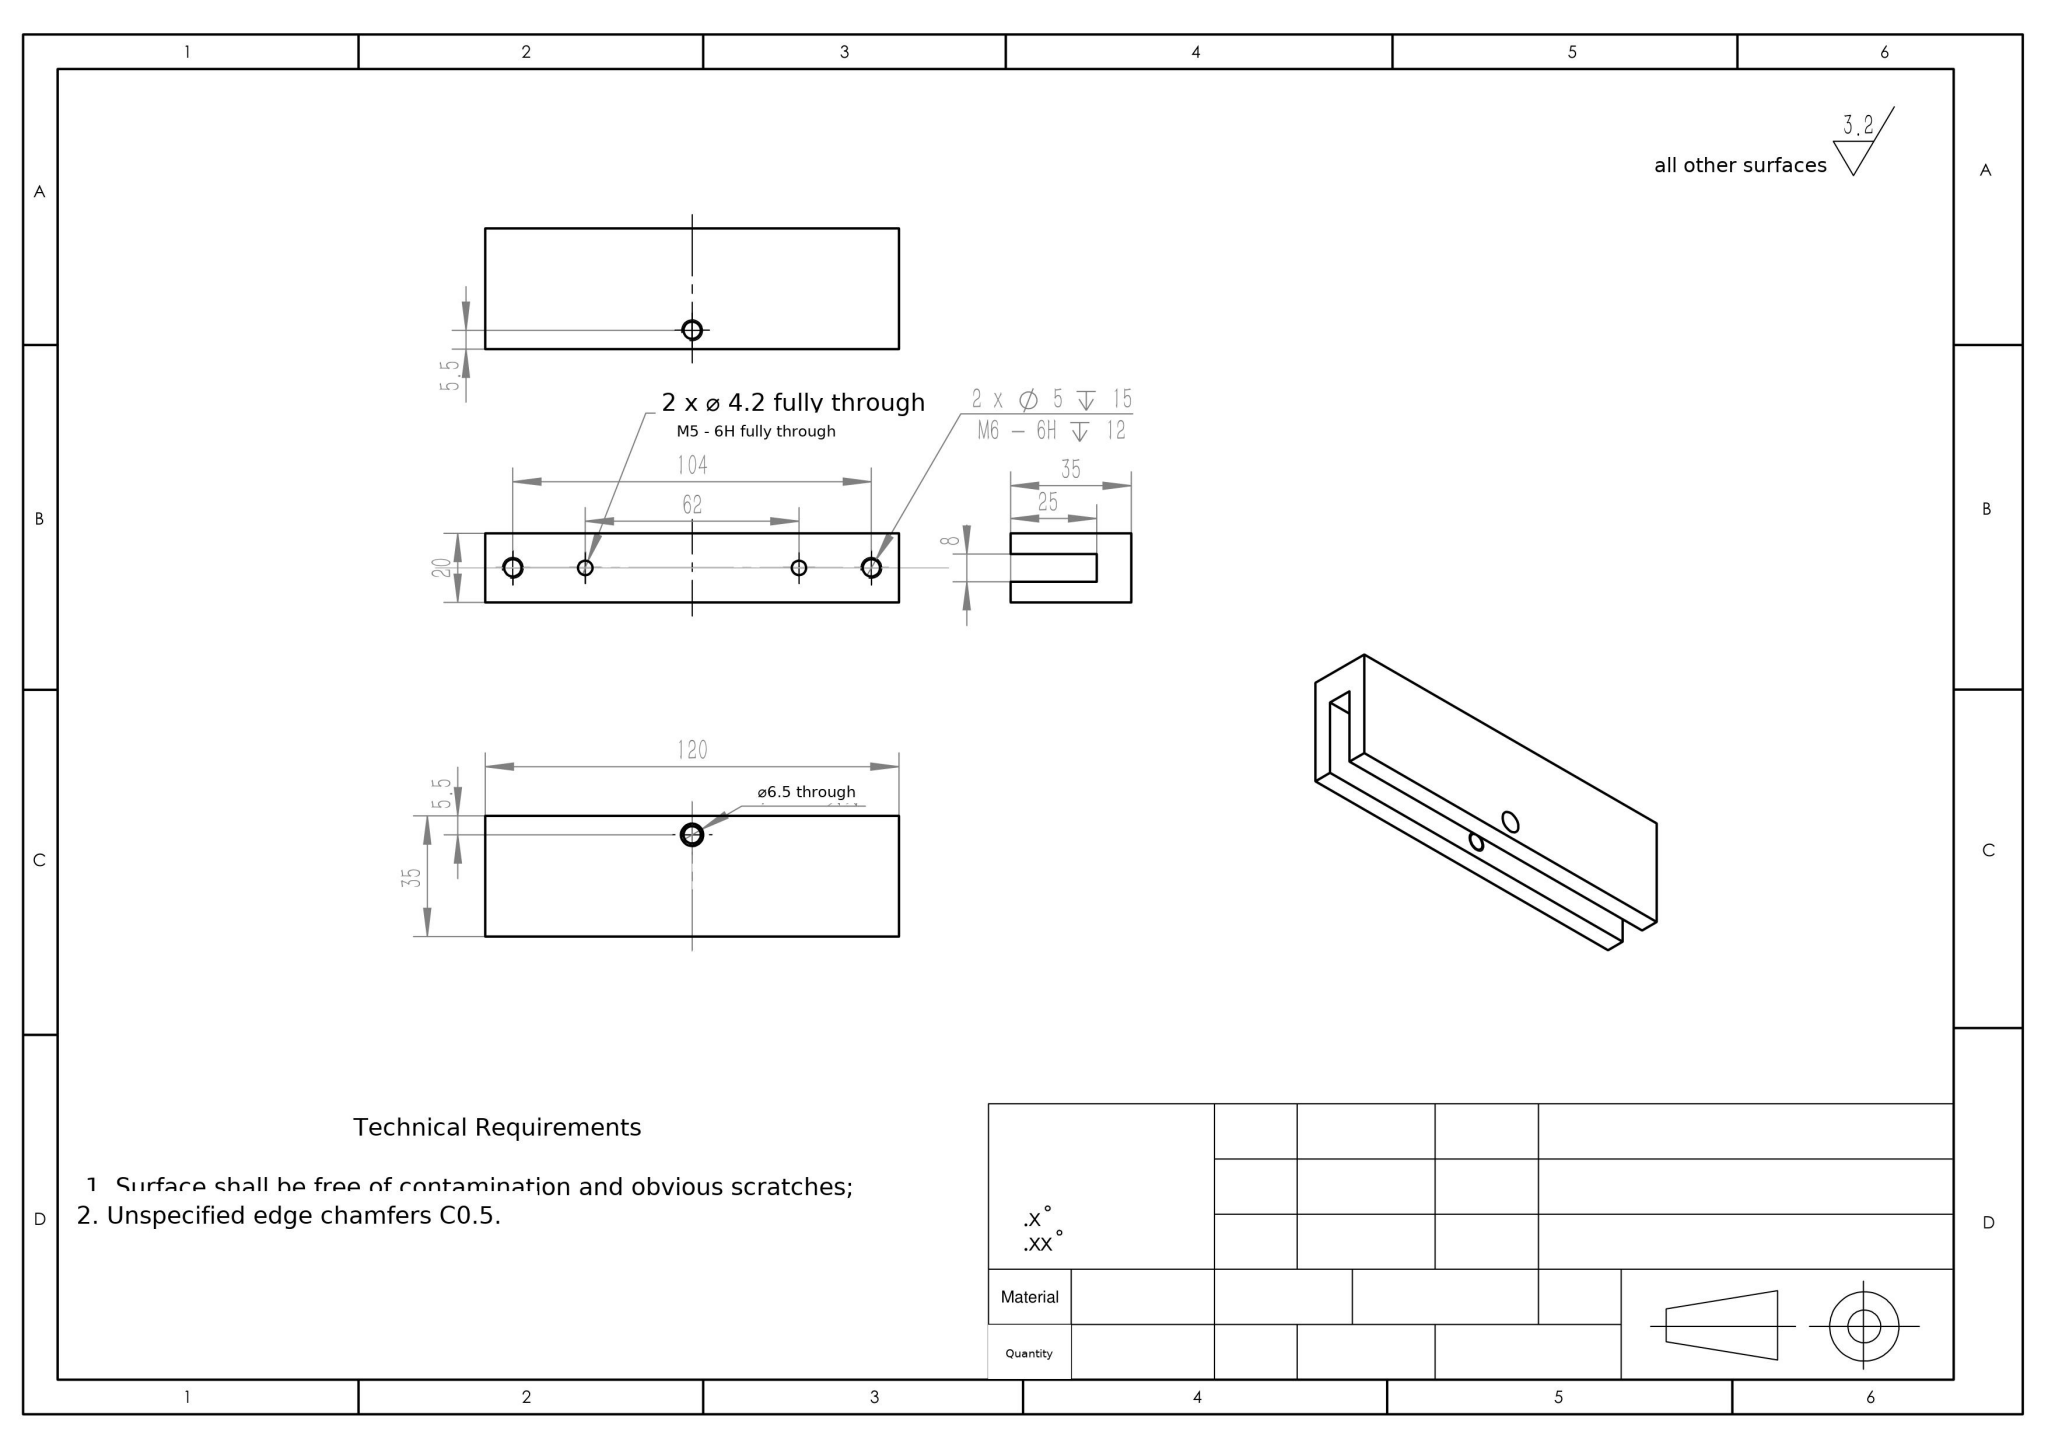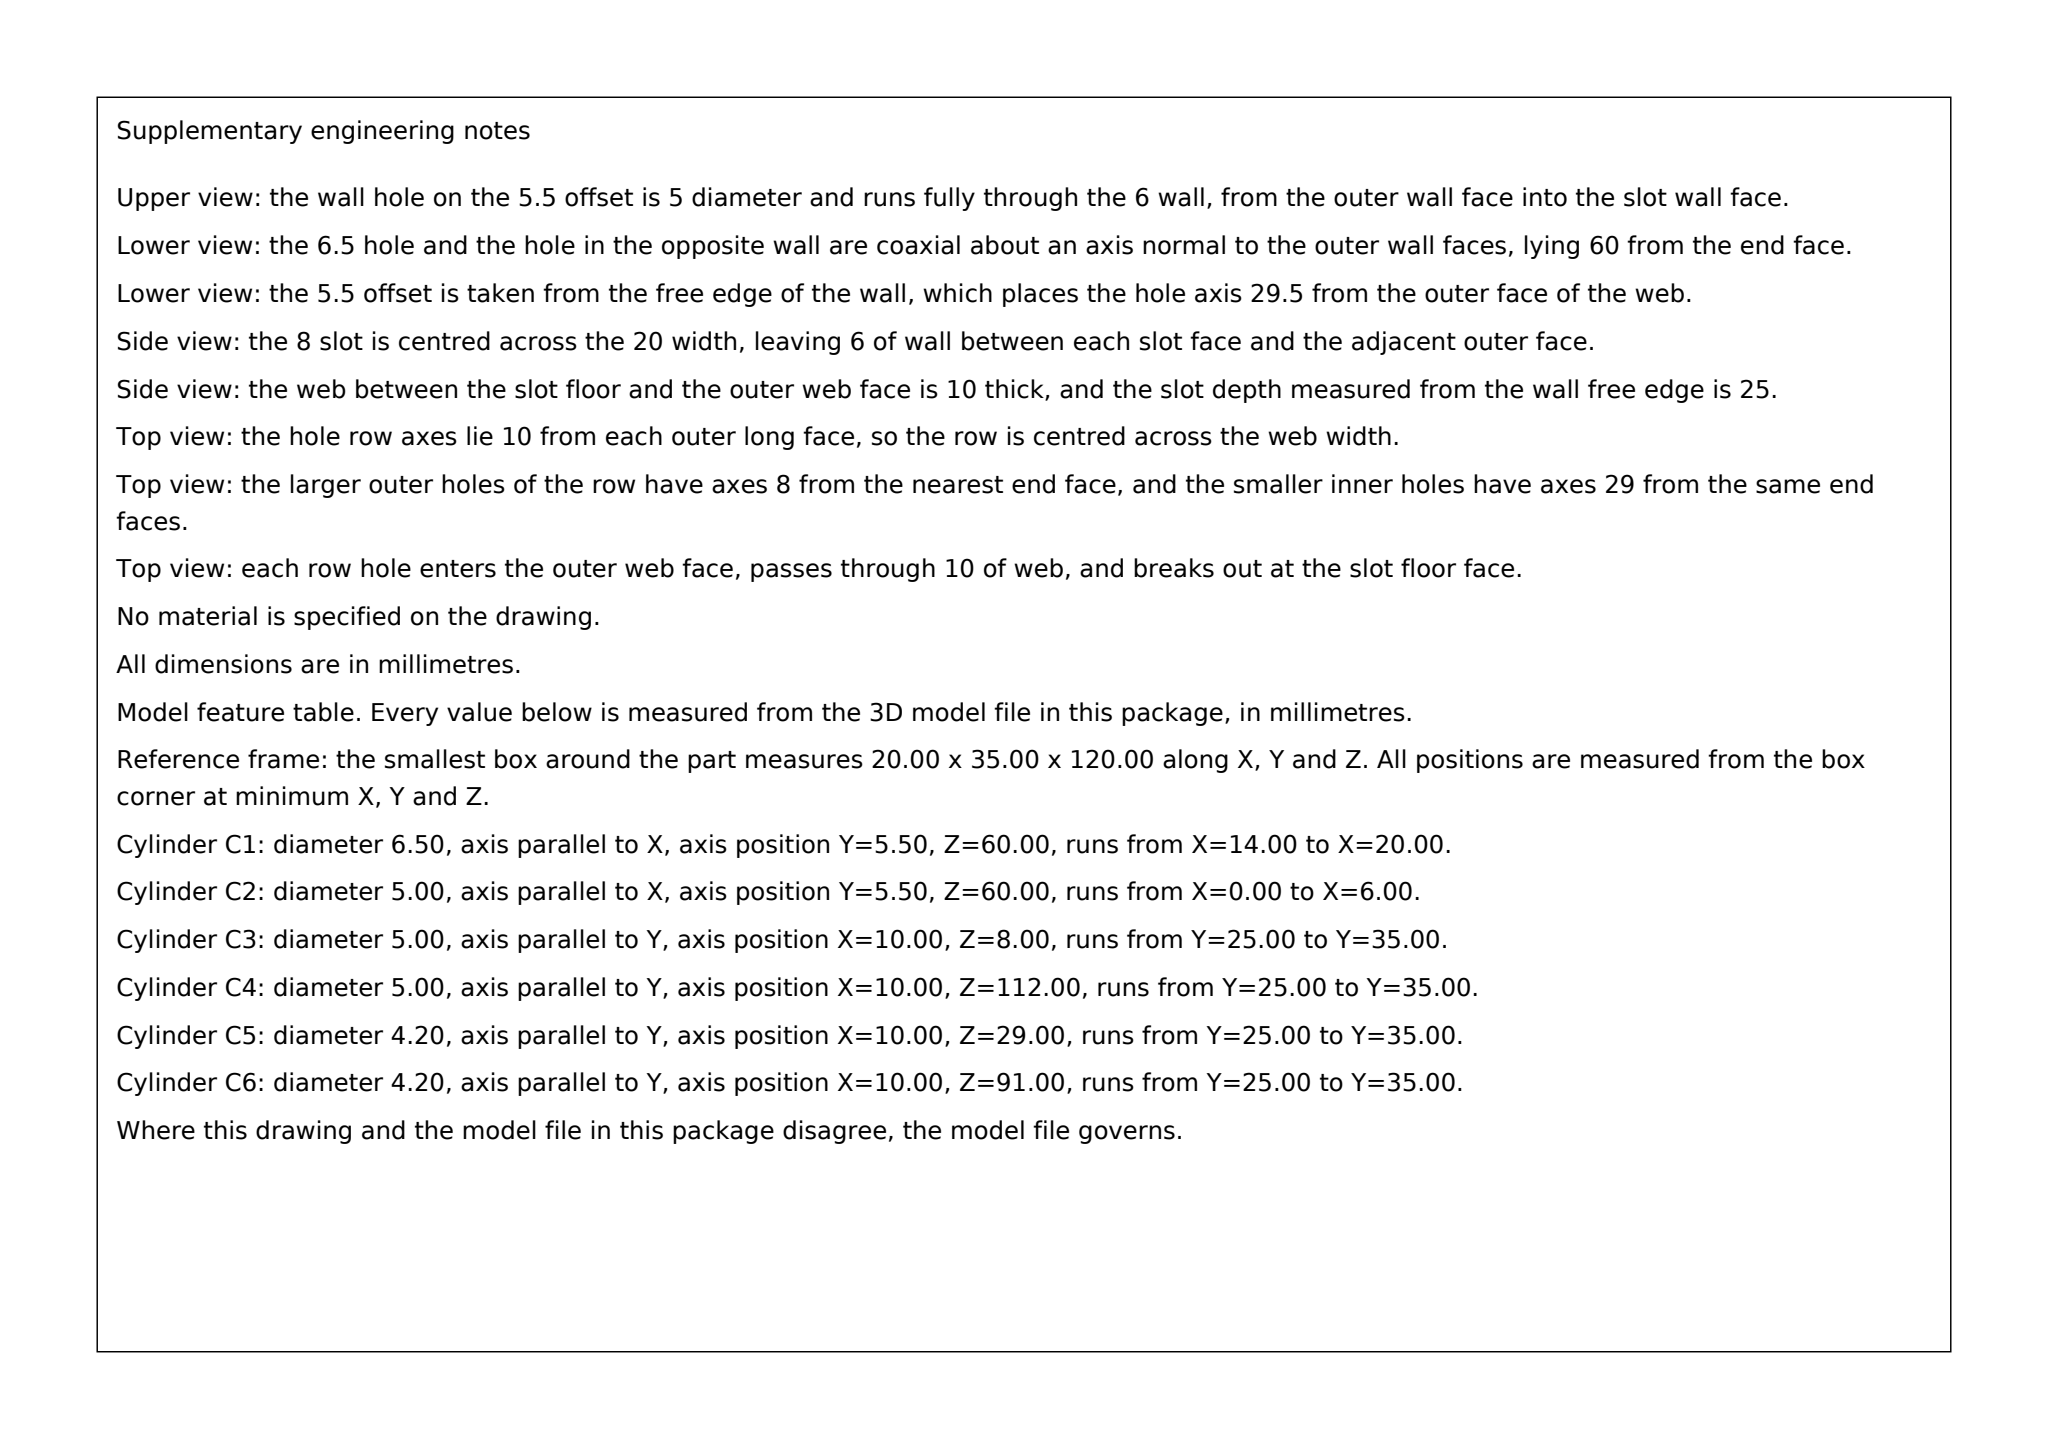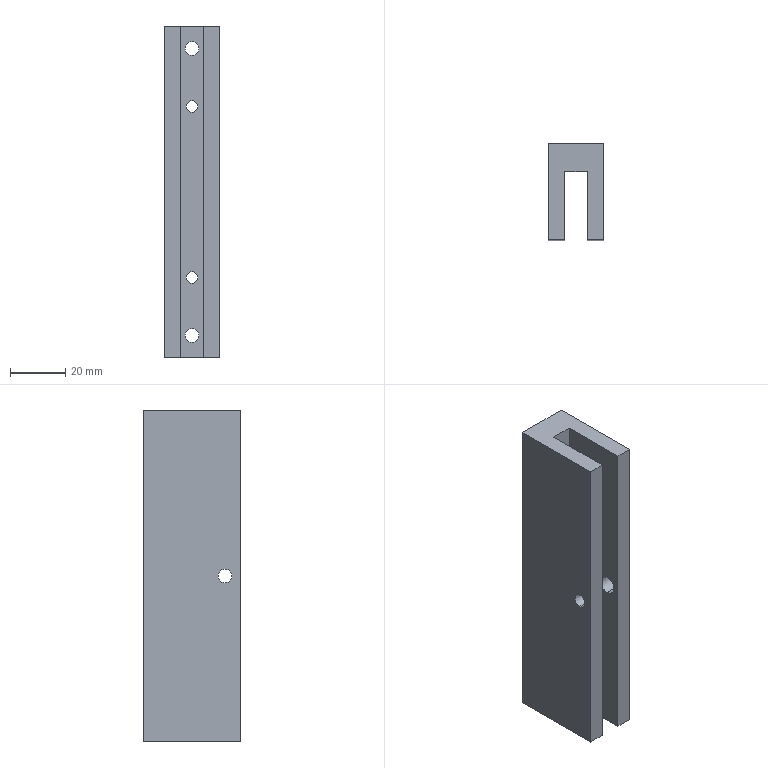Part | SolidWorks | mm | 1 solid | 22 faces | box 20 x 35 x 120 mm | volume 59013 mm3 | cylinder 12 | plane 10 | commonest cylinder face diameters 5 x6 4.2 x4 6.5 x2
build123d program:
from build123d import *

# Parameters (mm, degrees)
BOSS_EXTRUDE1_DEPTH   = 60
M5_TAPPED_HOLE1_D     = 4.2
M6_TAPPED_HOLE1_D     = 5
M6_TAPPED_HOLE1_DEPTH = 15
M6_TAPPED_HOLE1_TIP   = 1.502
CUT_EXTRUDE1_REACH    = 74.284
SKETCH6_R             = 3.25
M6_TAPPED_HOLE2_D     = 5
M6_TAPPED_HOLE2_DEPTH = 15
M6_TAPPED_HOLE2_TIP   = 1.502


with BuildPart() as part:
    # Sketch1 → Boss-Extrude1 (new, symmetric)
    with BuildSketch(Plane.XY):
        Polygon((20, 0), (0, 0), (0, -35), (6, -35), (6, -10), (14, -10), (14, -35), (20, -35), align=None)
    extrude(amount=BOSS_EXTRUDE1_DEPTH, both=True)

    # M5 Tapped Hole1 (through all)
    with Locations(Plane(origin=(0, -10, 0), x_dir=(-1, 0, 0), z_dir=(0, -1, 0))):
        with Locations((-10, -31), (-10, 31)):
            Hole(M5_TAPPED_HOLE1_D / 2)

    # M6 Tapped Hole1
    with Locations(Plane(origin=(0, 0, 0), x_dir=(1, 0, 0), z_dir=(0, 1, 0))):
        with Locations((10, 52), (10, -52)):
            Hole(M6_TAPPED_HOLE1_D / 2, depth=M6_TAPPED_HOLE1_DEPTH)
            with Locations((0, 0, -(M6_TAPPED_HOLE1_DEPTH + M6_TAPPED_HOLE1_TIP / 2))):  # 118° drill point
                Cone(0, M6_TAPPED_HOLE1_D / 2, M6_TAPPED_HOLE1_TIP, mode=Mode.SUBTRACT)

    # Sketch6 → Cut-Extrude1 (cut, up to next)
    with BuildSketch(Plane(origin=(20, 0, 0), x_dir=(0, 0, -1), z_dir=(1, 0, 0)), mode=Mode.PRIVATE) as cut_extrude1_sk1:
        with Locations((0, -29.5)):
            Circle(SKETCH6_R)
    cut_extrude1_tool1 = extrude(cut_extrude1_sk1.sketch, amount=-CUT_EXTRUDE1_REACH, mode=Mode.PRIVATE) & part.part
    add(cut_extrude1_tool1.solids().sort_by_distance((20, -29.5, 0))[0], mode=Mode.SUBTRACT)

    # M6 Tapped Hole2
    with Locations(Plane(origin=(6, 0, 0), x_dir=(0, 0, -1), z_dir=(1, 0, 0))):
        with Locations((0, -29.5)):
            Hole(M6_TAPPED_HOLE2_D / 2, depth=M6_TAPPED_HOLE2_DEPTH)
            with Locations((0, 0, -(M6_TAPPED_HOLE2_DEPTH + M6_TAPPED_HOLE2_TIP / 2))):  # 118° drill point
                Cone(0, M6_TAPPED_HOLE2_D / 2, M6_TAPPED_HOLE2_TIP, mode=Mode.SUBTRACT)


solid = part.part
STEP:
#1=CARTESIAN_POINT('',(0.,-29.5,2.5));
#2=VERTEX_POINT('',#1);
#3=CARTESIAN_POINT('',(0.,-29.5,-2.5));
#4=VERTEX_POINT('',#3);
#5=CARTESIAN_POINT('',(0.,-29.5,-0.));
#6=DIRECTION('',(1.,0.,0.));
#7=DIRECTION('',(0.,0.,-1.));
#8=AXIS2_PLACEMENT_3D('',#5,#6,#7);
#9=CIRCLE('',#8,2.5);
#10=EDGE_CURVE('',#2,#4,#9,.T.);
#11=ORIENTED_EDGE('',*,*,#10,.F.);
#12=CARTESIAN_POINT('',(6.,-29.5,2.5));
#13=VERTEX_POINT('',#12);
#14=CARTESIAN_POINT('',(6.,-29.5,2.5));
#15=DIRECTION('',(1.,0.,0.));
#16=VECTOR('',#15,1000.);
#17=LINE('',#14,#16);
#18=EDGE_CURVE('',#2,#13,#17,.T.);
#19=ORIENTED_EDGE('',*,*,#18,.T.);
#20=CARTESIAN_POINT('',(6.,-29.5,-2.5));
#21=VERTEX_POINT('',#20);
#22=CARTESIAN_POINT('',(6.,-29.5,-0.));
#23=DIRECTION('',(1.,0.,0.));
#24=DIRECTION('',(0.,0.,-1.));
#25=AXIS2_PLACEMENT_3D('',#22,#23,#24);
#26=CIRCLE('',#25,2.5);
#27=EDGE_CURVE('',#13,#21,#26,.T.);
#28=ORIENTED_EDGE('',*,*,#27,.T.);
#29=CARTESIAN_POINT('',(6.,-29.5,-2.5));
#30=DIRECTION('',(1.,0.,0.));
#31=VECTOR('',#30,1000.);
#32=LINE('',#29,#31);
#33=EDGE_CURVE('',#4,#21,#32,.T.);
#34=ORIENTED_EDGE('',*,*,#33,.F.);
#35=EDGE_LOOP('',(#11,#19,#28,#34));
#36=FACE_OUTER_BOUND('',#35,.T.);
#37=CARTESIAN_POINT('',(6.,-29.5,-0.));
#38=DIRECTION('',(1.,0.,0.));
#39=DIRECTION('',(0.,0.,-1.));
#40=AXIS2_PLACEMENT_3D('',#37,#38,#39);
#41=CYLINDRICAL_SURFACE('',#40,2.5);
#42=ADVANCED_FACE('',(#36),#41,.F.);
#43=CARTESIAN_POINT('',(14.,-29.5,-3.25));
#44=VERTEX_POINT('',#43);
#45=CARTESIAN_POINT('',(14.,-29.5,3.25));
#46=VERTEX_POINT('',#45);
#47=CARTESIAN_POINT('',(14.,-29.5,-0.));
#48=DIRECTION('',(-1.,-0.,0.));
#49=DIRECTION('',(0.,1.,0.));
#50=AXIS2_PLACEMENT_3D('',#47,#48,#49);
#51=CIRCLE('',#50,3.25);
#52=EDGE_CURVE('',#44,#46,#51,.T.);
#53=ORIENTED_EDGE('',*,*,#52,.T.);
#54=CARTESIAN_POINT('',(20.,-29.5,3.25));
#55=VERTEX_POINT('',#54);
#56=CARTESIAN_POINT('',(-0.001,-29.5,3.25));
#57=DIRECTION('',(1.,0.,0.));
#58=VECTOR('',#57,1000.);
#59=LINE('',#56,#58);
#60=EDGE_CURVE('',#46,#55,#59,.T.);
#61=ORIENTED_EDGE('',*,*,#60,.T.);
#62=CARTESIAN_POINT('',(20.,-29.5,-3.25));
#63=VERTEX_POINT('',#62);
#64=CARTESIAN_POINT('',(20.,-29.5,-0.));
#65=DIRECTION('',(1.,0.,0.));
#66=DIRECTION('',(0.,0.,-1.));
#67=AXIS2_PLACEMENT_3D('',#64,#65,#66);
#68=CIRCLE('',#67,3.25);
#69=EDGE_CURVE('',#55,#63,#68,.T.);
#70=ORIENTED_EDGE('',*,*,#69,.T.);
#71=CARTESIAN_POINT('',(-0.001,-29.5,-3.25));
#72=DIRECTION('',(1.,0.,0.));
#73=VECTOR('',#72,1000.);
#74=LINE('',#71,#73);
#75=EDGE_CURVE('',#44,#63,#74,.T.);
#76=ORIENTED_EDGE('',*,*,#75,.F.);
#77=EDGE_LOOP('',(#53,#61,#70,#76));
#78=FACE_OUTER_BOUND('',#77,.T.);
#79=CARTESIAN_POINT('',(-0.001,-29.5,-0.));
#80=DIRECTION('',(1.,0.,0.));
#81=DIRECTION('',(0.,0.,-1.));
#82=AXIS2_PLACEMENT_3D('',#79,#80,#81);
#83=CYLINDRICAL_SURFACE('',#82,3.25);
#84=ADVANCED_FACE('',(#78),#83,.F.);
#85=CARTESIAN_POINT('',(10.,-10.,-54.5));
#86=VERTEX_POINT('',#85);
#87=CARTESIAN_POINT('',(10.,-10.,-49.5));
#88=VERTEX_POINT('',#87);
#89=CARTESIAN_POINT('',(10.,-10.,-52.));
#90=DIRECTION('',(0.,1.,0.));
#91=DIRECTION('',(0.,0.,1.));
#92=AXIS2_PLACEMENT_3D('',#89,#90,#91);
#93=CIRCLE('',#92,2.5);
#94=EDGE_CURVE('',#86,#88,#93,.T.);
#95=ORIENTED_EDGE('',*,*,#94,.F.);
#96=CARTESIAN_POINT('',(10.,0.,-54.5));
#97=VERTEX_POINT('',#96);
#98=CARTESIAN_POINT('',(10.,0.,-54.5));
#99=DIRECTION('',(0.,1.,0.));
#100=VECTOR('',#99,1000.);
#101=LINE('',#98,#100);
#102=EDGE_CURVE('',#86,#97,#101,.T.);
#103=ORIENTED_EDGE('',*,*,#102,.T.);
#104=CARTESIAN_POINT('',(10.,0.,-49.5));
#105=VERTEX_POINT('',#104);
#106=CARTESIAN_POINT('',(10.,0.,-52.));
#107=DIRECTION('',(0.,1.,0.));
#108=DIRECTION('',(0.,0.,1.));
#109=AXIS2_PLACEMENT_3D('',#106,#107,#108);
#110=CIRCLE('',#109,2.5);
#111=EDGE_CURVE('',#97,#105,#110,.T.);
#112=ORIENTED_EDGE('',*,*,#111,.T.);
#113=CARTESIAN_POINT('',(10.,0.,-49.5));
#114=DIRECTION('',(0.,1.,0.));
#115=VECTOR('',#114,1000.);
#116=LINE('',#113,#115);
#117=EDGE_CURVE('',#88,#105,#116,.T.);
#118=ORIENTED_EDGE('',*,*,#117,.F.);
#119=EDGE_LOOP('',(#95,#103,#112,#118));
#120=FACE_OUTER_BOUND('',#119,.T.);
#121=CARTESIAN_POINT('',(10.,0.,-52.));
#122=DIRECTION('',(0.,1.,0.));
#123=DIRECTION('',(0.,0.,1.));
#124=AXIS2_PLACEMENT_3D('',#121,#122,#123);
#125=CYLINDRICAL_SURFACE('',#124,2.5);
#126=ADVANCED_FACE('',(#120),#125,.F.);
#127=CARTESIAN_POINT('',(10.,-10.,49.5));
#128=VERTEX_POINT('',#127);
#129=CARTESIAN_POINT('',(10.,-10.,54.5));
#130=VERTEX_POINT('',#129);
#131=CARTESIAN_POINT('',(10.,-10.,52.));
#132=DIRECTION('',(0.,1.,0.));
#133=DIRECTION('',(0.,0.,1.));
#134=AXIS2_PLACEMENT_3D('',#131,#132,#133);
#135=CIRCLE('',#134,2.5);
#136=EDGE_CURVE('',#128,#130,#135,.T.);
#137=ORIENTED_EDGE('',*,*,#136,.F.);
#138=CARTESIAN_POINT('',(10.,0.,49.5));
#139=VERTEX_POINT('',#138);
#140=CARTESIAN_POINT('',(10.,0.,49.5));
#141=DIRECTION('',(0.,1.,0.));
#142=VECTOR('',#141,1000.);
#143=LINE('',#140,#142);
#144=EDGE_CURVE('',#128,#139,#143,.T.);
#145=ORIENTED_EDGE('',*,*,#144,.T.);
#146=CARTESIAN_POINT('',(10.,0.,54.5));
#147=VERTEX_POINT('',#146);
#148=CARTESIAN_POINT('',(10.,0.,52.));
#149=DIRECTION('',(0.,1.,0.));
#150=DIRECTION('',(0.,0.,1.));
#151=AXIS2_PLACEMENT_3D('',#148,#149,#150);
#152=CIRCLE('',#151,2.5);
#153=EDGE_CURVE('',#139,#147,#152,.T.);
#154=ORIENTED_EDGE('',*,*,#153,.T.);
#155=CARTESIAN_POINT('',(10.,0.,54.5));
#156=DIRECTION('',(0.,1.,0.));
#157=VECTOR('',#156,1000.);
#158=LINE('',#155,#157);
#159=EDGE_CURVE('',#130,#147,#158,.T.);
#160=ORIENTED_EDGE('',*,*,#159,.F.);
#161=EDGE_LOOP('',(#137,#145,#154,#160));
#162=FACE_OUTER_BOUND('',#161,.T.);
#163=CARTESIAN_POINT('',(10.,0.,52.));
#164=DIRECTION('',(0.,1.,0.));
#165=DIRECTION('',(0.,0.,1.));
#166=AXIS2_PLACEMENT_3D('',#163,#164,#165);
#167=CYLINDRICAL_SURFACE('',#166,2.5);
#168=ADVANCED_FACE('',(#162),#167,.F.);
#169=CARTESIAN_POINT('',(10.,0.,33.1));
#170=VERTEX_POINT('',#169);
#171=CARTESIAN_POINT('',(10.,0.,28.9));
#172=VERTEX_POINT('',#171);
#173=CARTESIAN_POINT('',(10.,0.,31.));
#174=DIRECTION('',(0.,-1.,0.));
#175=DIRECTION('',(0.,0.,-1.));
#176=AXIS2_PLACEMENT_3D('',#173,#174,#175);
#177=CIRCLE('',#176,2.1);
#178=EDGE_CURVE('',#170,#172,#177,.T.);
#179=ORIENTED_EDGE('',*,*,#178,.F.);
#180=CARTESIAN_POINT('',(10.,-10.,33.1));
#181=VERTEX_POINT('',#180);
#182=CARTESIAN_POINT('',(10.,-10.,33.1));
#183=DIRECTION('',(0.,-1.,0.));
#184=VECTOR('',#183,1000.);
#185=LINE('',#182,#184);
#186=EDGE_CURVE('',#170,#181,#185,.T.);
#187=ORIENTED_EDGE('',*,*,#186,.T.);
#188=CARTESIAN_POINT('',(10.,-10.,28.9));
#189=VERTEX_POINT('',#188);
#190=CARTESIAN_POINT('',(10.,-10.,31.));
#191=DIRECTION('',(0.,-1.,0.));
#192=DIRECTION('',(0.,0.,-1.));
#193=AXIS2_PLACEMENT_3D('',#190,#191,#192);
#194=CIRCLE('',#193,2.1);
#195=EDGE_CURVE('',#181,#189,#194,.T.);
#196=ORIENTED_EDGE('',*,*,#195,.T.);
#197=CARTESIAN_POINT('',(10.,-10.,28.9));
#198=DIRECTION('',(0.,-1.,0.));
#199=VECTOR('',#198,1000.);
#200=LINE('',#197,#199);
#201=EDGE_CURVE('',#172,#189,#200,.T.);
#202=ORIENTED_EDGE('',*,*,#201,.F.);
#203=EDGE_LOOP('',(#179,#187,#196,#202));
#204=FACE_OUTER_BOUND('',#203,.T.);
#205=CARTESIAN_POINT('',(10.,-10.,31.));
#206=DIRECTION('',(0.,-1.,0.));
#207=DIRECTION('',(0.,0.,-1.));
#208=AXIS2_PLACEMENT_3D('',#205,#206,#207);
#209=CYLINDRICAL_SURFACE('',#208,2.1);
#210=ADVANCED_FACE('',(#204),#209,.F.);
#211=CARTESIAN_POINT('',(10.,0.,-28.9));
#212=VERTEX_POINT('',#211);
#213=CARTESIAN_POINT('',(10.,0.,-33.1));
#214=VERTEX_POINT('',#213);
#215=CARTESIAN_POINT('',(10.,0.,-31.));
#216=DIRECTION('',(0.,-1.,0.));
#217=DIRECTION('',(0.,0.,-1.));
#218=AXIS2_PLACEMENT_3D('',#215,#216,#217);
#219=CIRCLE('',#218,2.1);
#220=EDGE_CURVE('',#212,#214,#219,.T.);
#221=ORIENTED_EDGE('',*,*,#220,.F.);
#222=CARTESIAN_POINT('',(10.,-10.,-28.9));
#223=VERTEX_POINT('',#222);
#224=CARTESIAN_POINT('',(10.,-10.,-28.9));
#225=DIRECTION('',(0.,-1.,0.));
#226=VECTOR('',#225,1000.);
#227=LINE('',#224,#226);
#228=EDGE_CURVE('',#212,#223,#227,.T.);
#229=ORIENTED_EDGE('',*,*,#228,.T.);
#230=CARTESIAN_POINT('',(10.,-10.,-33.1));
#231=VERTEX_POINT('',#230);
#232=CARTESIAN_POINT('',(10.,-10.,-31.));
#233=DIRECTION('',(0.,-1.,0.));
#234=DIRECTION('',(0.,0.,-1.));
#235=AXIS2_PLACEMENT_3D('',#232,#233,#234);
#236=CIRCLE('',#235,2.1);
#237=EDGE_CURVE('',#223,#231,#236,.T.);
#238=ORIENTED_EDGE('',*,*,#237,.T.);
#239=CARTESIAN_POINT('',(10.,-10.,-33.1));
#240=DIRECTION('',(0.,-1.,0.));
#241=VECTOR('',#240,1000.);
#242=LINE('',#239,#241);
#243=EDGE_CURVE('',#214,#231,#242,.T.);
#244=ORIENTED_EDGE('',*,*,#243,.F.);
#245=EDGE_LOOP('',(#221,#229,#238,#244));
#246=FACE_OUTER_BOUND('',#245,.T.);
#247=CARTESIAN_POINT('',(10.,-10.,-31.));
#248=DIRECTION('',(0.,-1.,0.));
#249=DIRECTION('',(0.,0.,-1.));
#250=AXIS2_PLACEMENT_3D('',#247,#248,#249);
#251=CYLINDRICAL_SURFACE('',#250,2.1);
#252=ADVANCED_FACE('',(#246),#251,.F.);
#253=CARTESIAN_POINT('',(20.,-29.5,-0.));
#254=DIRECTION('',(1.,0.,0.));
#255=DIRECTION('',(0.,0.,-1.));
#256=AXIS2_PLACEMENT_3D('',#253,#254,#255);
#257=CIRCLE('',#256,3.25);
#258=EDGE_CURVE('',#63,#55,#257,.T.);
#259=ORIENTED_EDGE('',*,*,#258,.F.);
#260=ORIENTED_EDGE('',*,*,#69,.F.);
#261=EDGE_LOOP('',(#259,#260));
#262=FACE_BOUND('',#261,.T.);
#263=CARTESIAN_POINT('',(20.,-35.,-60.));
#264=VERTEX_POINT('',#263);
#265=CARTESIAN_POINT('',(20.,-0.,-60.));
#266=VERTEX_POINT('',#265);
#267=CARTESIAN_POINT('',(20.,-35.,-60.));
#268=DIRECTION('',(0.,1.,0.));
#269=VECTOR('',#268,1000.);
#270=LINE('',#267,#269);
#271=EDGE_CURVE('',#264,#266,#270,.T.);
#272=ORIENTED_EDGE('',*,*,#271,.T.);
#273=CARTESIAN_POINT('',(20.,-0.,60.));
#274=VERTEX_POINT('',#273);
#275=CARTESIAN_POINT('',(20.,-0.,60.));
#276=DIRECTION('',(0.,0.,-1.));
#277=VECTOR('',#276,1000.);
#278=LINE('',#275,#277);
#279=EDGE_CURVE('',#274,#266,#278,.T.);
#280=ORIENTED_EDGE('',*,*,#279,.F.);
#281=CARTESIAN_POINT('',(20.,-35.,60.));
#282=VERTEX_POINT('',#281);
#283=CARTESIAN_POINT('',(20.,-35.,60.));
#284=DIRECTION('',(0.,1.,0.));
#285=VECTOR('',#284,1000.);
#286=LINE('',#283,#285);
#287=EDGE_CURVE('',#282,#274,#286,.T.);
#288=ORIENTED_EDGE('',*,*,#287,.F.);
#289=CARTESIAN_POINT('',(20.,-35.,60.));
#290=DIRECTION('',(0.,0.,-1.));
#291=VECTOR('',#290,1000.);
#292=LINE('',#289,#291);
#293=EDGE_CURVE('',#282,#264,#292,.T.);
#294=ORIENTED_EDGE('',*,*,#293,.T.);
#295=EDGE_LOOP('',(#272,#280,#288,#294));
#296=FACE_OUTER_BOUND('',#295,.T.);
#297=CARTESIAN_POINT('',(20.,-35.,60.));
#298=DIRECTION('',(-1.,0.,0.));
#299=DIRECTION('',(0.,0.,1.));
#300=AXIS2_PLACEMENT_3D('',#297,#298,#299);
#301=PLANE('',#300);
#302=ADVANCED_FACE('',(#262,#296),#301,.F.);
#303=CARTESIAN_POINT('',(10.,0.,-52.));
#304=DIRECTION('',(0.,1.,0.));
#305=DIRECTION('',(0.,0.,1.));
#306=AXIS2_PLACEMENT_3D('',#303,#304,#305);
#307=CIRCLE('',#306,2.5);
#308=EDGE_CURVE('',#105,#97,#307,.T.);
#309=ORIENTED_EDGE('',*,*,#308,.F.);
#310=ORIENTED_EDGE('',*,*,#111,.F.);
#311=EDGE_LOOP('',(#309,#310));
#312=FACE_BOUND('',#311,.T.);
#313=CARTESIAN_POINT('',(10.,0.,52.));
#314=DIRECTION('',(0.,1.,0.));
#315=DIRECTION('',(0.,0.,1.));
#316=AXIS2_PLACEMENT_3D('',#313,#314,#315);
#317=CIRCLE('',#316,2.5);
#318=EDGE_CURVE('',#147,#139,#317,.T.);
#319=ORIENTED_EDGE('',*,*,#318,.F.);
#320=ORIENTED_EDGE('',*,*,#153,.F.);
#321=EDGE_LOOP('',(#319,#320));
#322=FACE_BOUND('',#321,.T.);
#323=CARTESIAN_POINT('',(10.,0.,31.));
#324=DIRECTION('',(0.,-1.,0.));
#325=DIRECTION('',(0.,0.,-1.));
#326=AXIS2_PLACEMENT_3D('',#323,#324,#325);
#327=CIRCLE('',#326,2.1);
#328=EDGE_CURVE('',#172,#170,#327,.T.);
#329=ORIENTED_EDGE('',*,*,#328,.T.);
#330=ORIENTED_EDGE('',*,*,#178,.T.);
#331=EDGE_LOOP('',(#329,#330));
#332=FACE_BOUND('',#331,.T.);
#333=CARTESIAN_POINT('',(10.,0.,-31.));
#334=DIRECTION('',(0.,-1.,0.));
#335=DIRECTION('',(0.,0.,-1.));
#336=AXIS2_PLACEMENT_3D('',#333,#334,#335);
#337=CIRCLE('',#336,2.1);
#338=EDGE_CURVE('',#214,#212,#337,.T.);
#339=ORIENTED_EDGE('',*,*,#338,.T.);
#340=ORIENTED_EDGE('',*,*,#220,.T.);
#341=EDGE_LOOP('',(#339,#340));
#342=FACE_BOUND('',#341,.T.);
#343=CARTESIAN_POINT('',(0.,0.,-60.));
#344=VERTEX_POINT('',#343);
#345=CARTESIAN_POINT('',(20.,-0.,-60.));
#346=DIRECTION('',(-1.,0.,0.));
#347=VECTOR('',#346,1000.);
#348=LINE('',#345,#347);
#349=EDGE_CURVE('',#266,#344,#348,.T.);
#350=ORIENTED_EDGE('',*,*,#349,.T.);
#351=CARTESIAN_POINT('',(0.,0.,60.));
#352=VERTEX_POINT('',#351);
#353=CARTESIAN_POINT('',(0.,0.,60.));
#354=DIRECTION('',(0.,0.,-1.));
#355=VECTOR('',#354,1000.);
#356=LINE('',#353,#355);
#357=EDGE_CURVE('',#352,#344,#356,.T.);
#358=ORIENTED_EDGE('',*,*,#357,.F.);
#359=CARTESIAN_POINT('',(20.,-0.,60.));
#360=DIRECTION('',(-1.,0.,0.));
#361=VECTOR('',#360,1000.);
#362=LINE('',#359,#361);
#363=EDGE_CURVE('',#274,#352,#362,.T.);
#364=ORIENTED_EDGE('',*,*,#363,.F.);
#365=ORIENTED_EDGE('',*,*,#279,.T.);
#366=EDGE_LOOP('',(#350,#358,#364,#365));
#367=FACE_OUTER_BOUND('',#366,.T.);
#368=CARTESIAN_POINT('',(20.,-0.,60.));
#369=DIRECTION('',(-0.,-1.,0.));
#370=DIRECTION('',(1.,-0.,0.));
#371=AXIS2_PLACEMENT_3D('',#368,#369,#370);
#372=PLANE('',#371);
#373=ADVANCED_FACE('',(#312,#322,#332,#342,#367),#372,.F.);
#374=CARTESIAN_POINT('',(0.,-29.5,-0.));
#375=DIRECTION('',(1.,0.,0.));
#376=DIRECTION('',(0.,0.,-1.));
#377=AXIS2_PLACEMENT_3D('',#374,#375,#376);
#378=CIRCLE('',#377,2.5);
#379=EDGE_CURVE('',#4,#2,#378,.T.);
#380=ORIENTED_EDGE('',*,*,#379,.T.);
#381=ORIENTED_EDGE('',*,*,#10,.T.);
#382=EDGE_LOOP('',(#380,#381));
#383=FACE_BOUND('',#382,.T.);
#384=CARTESIAN_POINT('',(0.,-35.,-60.));
#385=VERTEX_POINT('',#384);
#386=CARTESIAN_POINT('',(0.,0.,-60.));
#387=DIRECTION('',(0.,-1.,0.));
#388=VECTOR('',#387,1000.);
#389=LINE('',#386,#388);
#390=EDGE_CURVE('',#344,#385,#389,.T.);
#391=ORIENTED_EDGE('',*,*,#390,.T.);
#392=CARTESIAN_POINT('',(0.,-35.,60.));
#393=VERTEX_POINT('',#392);
#394=CARTESIAN_POINT('',(0.,-35.,60.));
#395=DIRECTION('',(0.,0.,-1.));
#396=VECTOR('',#395,1000.);
#397=LINE('',#394,#396);
#398=EDGE_CURVE('',#393,#385,#397,.T.);
#399=ORIENTED_EDGE('',*,*,#398,.F.);
#400=CARTESIAN_POINT('',(0.,0.,60.));
#401=DIRECTION('',(0.,-1.,0.));
#402=VECTOR('',#401,1000.);
#403=LINE('',#400,#402);
#404=EDGE_CURVE('',#352,#393,#403,.T.);
#405=ORIENTED_EDGE('',*,*,#404,.F.);
#406=ORIENTED_EDGE('',*,*,#357,.T.);
#407=EDGE_LOOP('',(#391,#399,#405,#406));
#408=FACE_OUTER_BOUND('',#407,.T.);
#409=CARTESIAN_POINT('',(0.,0.,60.));
#410=DIRECTION('',(1.,0.,0.));
#411=DIRECTION('',(0.,0.,-1.));
#412=AXIS2_PLACEMENT_3D('',#409,#410,#411);
#413=PLANE('',#412);
#414=ADVANCED_FACE('',(#383,#408),#413,.F.);
#415=CARTESIAN_POINT('',(6.,-35.,-60.));
#416=VERTEX_POINT('',#415);
#417=CARTESIAN_POINT('',(0.,-35.,-60.));
#418=DIRECTION('',(1.,0.,0.));
#419=VECTOR('',#418,1000.);
#420=LINE('',#417,#419);
#421=EDGE_CURVE('',#385,#416,#420,.T.);
#422=ORIENTED_EDGE('',*,*,#421,.T.);
#423=CARTESIAN_POINT('',(6.,-35.,60.));
#424=VERTEX_POINT('',#423);
#425=CARTESIAN_POINT('',(6.,-35.,60.));
#426=DIRECTION('',(0.,0.,-1.));
#427=VECTOR('',#426,1000.);
#428=LINE('',#425,#427);
#429=EDGE_CURVE('',#424,#416,#428,.T.);
#430=ORIENTED_EDGE('',*,*,#429,.F.);
#431=CARTESIAN_POINT('',(0.,-35.,60.));
#432=DIRECTION('',(1.,0.,0.));
#433=VECTOR('',#432,1000.);
#434=LINE('',#431,#433);
#435=EDGE_CURVE('',#393,#424,#434,.T.);
#436=ORIENTED_EDGE('',*,*,#435,.F.);
#437=ORIENTED_EDGE('',*,*,#398,.T.);
#438=EDGE_LOOP('',(#422,#430,#436,#437));
#439=FACE_OUTER_BOUND('',#438,.T.);
#440=CARTESIAN_POINT('',(0.,-35.,60.));
#441=DIRECTION('',(0.,1.,0.));
#442=DIRECTION('',(0.,0.,1.));
#443=AXIS2_PLACEMENT_3D('',#440,#441,#442);
#444=PLANE('',#443);
#445=ADVANCED_FACE('',(#439),#444,.F.);
#446=CARTESIAN_POINT('',(6.,-29.5,-0.));
#447=DIRECTION('',(1.,0.,0.));
#448=DIRECTION('',(0.,0.,-1.));
#449=AXIS2_PLACEMENT_3D('',#446,#447,#448);
#450=CIRCLE('',#449,2.5);
#451=EDGE_CURVE('',#21,#13,#450,.T.);
#452=ORIENTED_EDGE('',*,*,#451,.F.);
#453=ORIENTED_EDGE('',*,*,#27,.F.);
#454=EDGE_LOOP('',(#452,#453));
#455=FACE_BOUND('',#454,.T.);
#456=CARTESIAN_POINT('',(6.,-10.,-60.));
#457=VERTEX_POINT('',#456);
#458=CARTESIAN_POINT('',(6.,-35.,-60.));
#459=DIRECTION('',(-0.,1.,0.));
#460=VECTOR('',#459,1000.);
#461=LINE('',#458,#460);
#462=EDGE_CURVE('',#416,#457,#461,.T.);
#463=ORIENTED_EDGE('',*,*,#462,.T.);
#464=CARTESIAN_POINT('',(6.,-10.,60.));
#465=VERTEX_POINT('',#464);
#466=CARTESIAN_POINT('',(6.,-10.,60.));
#467=DIRECTION('',(0.,0.,-1.));
#468=VECTOR('',#467,1000.);
#469=LINE('',#466,#468);
#470=EDGE_CURVE('',#465,#457,#469,.T.);
#471=ORIENTED_EDGE('',*,*,#470,.F.);
#472=CARTESIAN_POINT('',(6.,-35.,60.));
#473=DIRECTION('',(-0.,1.,0.));
#474=VECTOR('',#473,1000.);
#475=LINE('',#472,#474);
#476=EDGE_CURVE('',#424,#465,#475,.T.);
#477=ORIENTED_EDGE('',*,*,#476,.F.);
#478=ORIENTED_EDGE('',*,*,#429,.T.);
#479=EDGE_LOOP('',(#463,#471,#477,#478));
#480=FACE_OUTER_BOUND('',#479,.T.);
#481=CARTESIAN_POINT('',(6.,-35.,60.));
#482=DIRECTION('',(-1.,-0.,0.));
#483=DIRECTION('',(0.,-1.,0.));
#484=AXIS2_PLACEMENT_3D('',#481,#482,#483);
#485=PLANE('',#484);
#486=ADVANCED_FACE('',(#455,#480),#485,.F.);
#487=CARTESIAN_POINT('',(10.,-10.,-52.));
#488=DIRECTION('',(0.,1.,0.));
#489=DIRECTION('',(0.,0.,1.));
#490=AXIS2_PLACEMENT_3D('',#487,#488,#489);
#491=CIRCLE('',#490,2.5);
#492=EDGE_CURVE('',#88,#86,#491,.T.);
#493=ORIENTED_EDGE('',*,*,#492,.T.);
#494=ORIENTED_EDGE('',*,*,#94,.T.);
#495=EDGE_LOOP('',(#493,#494));
#496=FACE_BOUND('',#495,.T.);
#497=CARTESIAN_POINT('',(10.,-10.,52.));
#498=DIRECTION('',(0.,1.,0.));
#499=DIRECTION('',(0.,0.,1.));
#500=AXIS2_PLACEMENT_3D('',#497,#498,#499);
#501=CIRCLE('',#500,2.5);
#502=EDGE_CURVE('',#130,#128,#501,.T.);
#503=ORIENTED_EDGE('',*,*,#502,.T.);
#504=ORIENTED_EDGE('',*,*,#136,.T.);
#505=EDGE_LOOP('',(#503,#504));
#506=FACE_BOUND('',#505,.T.);
#507=CARTESIAN_POINT('',(10.,-10.,31.));
#508=DIRECTION('',(0.,-1.,0.));
#509=DIRECTION('',(0.,0.,-1.));
#510=AXIS2_PLACEMENT_3D('',#507,#508,#509);
#511=CIRCLE('',#510,2.1);
#512=EDGE_CURVE('',#189,#181,#511,.T.);
#513=ORIENTED_EDGE('',*,*,#512,.F.);
#514=ORIENTED_EDGE('',*,*,#195,.F.);
#515=EDGE_LOOP('',(#513,#514));
#516=FACE_BOUND('',#515,.T.);
#517=CARTESIAN_POINT('',(10.,-10.,-31.));
#518=DIRECTION('',(0.,-1.,0.));
#519=DIRECTION('',(0.,0.,-1.));
#520=AXIS2_PLACEMENT_3D('',#517,#518,#519);
#521=CIRCLE('',#520,2.1);
#522=EDGE_CURVE('',#231,#223,#521,.T.);
#523=ORIENTED_EDGE('',*,*,#522,.F.);
#524=ORIENTED_EDGE('',*,*,#237,.F.);
#525=EDGE_LOOP('',(#523,#524));
#526=FACE_BOUND('',#525,.T.);
#527=CARTESIAN_POINT('',(14.,-10.,-60.));
#528=VERTEX_POINT('',#527);
#529=CARTESIAN_POINT('',(6.,-10.,-60.));
#530=DIRECTION('',(1.,0.,0.));
#531=VECTOR('',#530,1000.);
#532=LINE('',#529,#531);
#533=EDGE_CURVE('',#457,#528,#532,.T.);
#534=ORIENTED_EDGE('',*,*,#533,.T.);
#535=CARTESIAN_POINT('',(14.,-10.,60.));
#536=VERTEX_POINT('',#535);
#537=CARTESIAN_POINT('',(14.,-10.,60.));
#538=DIRECTION('',(0.,0.,-1.));
#539=VECTOR('',#538,1000.);
#540=LINE('',#537,#539);
#541=EDGE_CURVE('',#536,#528,#540,.T.);
#542=ORIENTED_EDGE('',*,*,#541,.F.);
#543=CARTESIAN_POINT('',(6.,-10.,60.));
#544=DIRECTION('',(1.,0.,0.));
#545=VECTOR('',#544,1000.);
#546=LINE('',#543,#545);
#547=EDGE_CURVE('',#465,#536,#546,.T.);
#548=ORIENTED_EDGE('',*,*,#547,.F.);
#549=ORIENTED_EDGE('',*,*,#470,.T.);
#550=EDGE_LOOP('',(#534,#542,#548,#549));
#551=FACE_OUTER_BOUND('',#550,.T.);
#552=CARTESIAN_POINT('',(6.,-10.,60.));
#553=DIRECTION('',(0.,1.,0.));
#554=DIRECTION('',(0.,0.,1.));
#555=AXIS2_PLACEMENT_3D('',#552,#553,#554);
#556=PLANE('',#555);
#557=ADVANCED_FACE('',(#496,#506,#516,#526,#551),#556,.F.);
#558=ORIENTED_EDGE('',*,*,#52,.F.);
#559=CARTESIAN_POINT('',(14.,-29.5,-0.));
#560=DIRECTION('',(-1.,-0.,0.));
#561=DIRECTION('',(0.,1.,0.));
#562=AXIS2_PLACEMENT_3D('',#559,#560,#561);
#563=CIRCLE('',#562,3.25);
#564=EDGE_CURVE('',#46,#44,#563,.T.);
#565=ORIENTED_EDGE('',*,*,#564,.F.);
#566=EDGE_LOOP('',(#558,#565));
#567=FACE_BOUND('',#566,.T.);
#568=CARTESIAN_POINT('',(14.,-35.,-60.));
#569=VERTEX_POINT('',#568);
#570=CARTESIAN_POINT('',(14.,-10.,-60.));
#571=DIRECTION('',(0.,-1.,0.));
#572=VECTOR('',#571,1000.);
#573=LINE('',#570,#572);
#574=EDGE_CURVE('',#528,#569,#573,.T.);
#575=ORIENTED_EDGE('',*,*,#574,.T.);
#576=CARTESIAN_POINT('',(14.,-35.,60.));
#577=VERTEX_POINT('',#576);
#578=CARTESIAN_POINT('',(14.,-35.,60.));
#579=DIRECTION('',(0.,0.,-1.));
#580=VECTOR('',#579,1000.);
#581=LINE('',#578,#580);
#582=EDGE_CURVE('',#577,#569,#581,.T.);
#583=ORIENTED_EDGE('',*,*,#582,.F.);
#584=CARTESIAN_POINT('',(14.,-10.,60.));
#585=DIRECTION('',(0.,-1.,0.));
#586=VECTOR('',#585,1000.);
#587=LINE('',#584,#586);
#588=EDGE_CURVE('',#536,#577,#587,.T.);
#589=ORIENTED_EDGE('',*,*,#588,.F.);
#590=ORIENTED_EDGE('',*,*,#541,.T.);
#591=EDGE_LOOP('',(#575,#583,#589,#590));
#592=FACE_OUTER_BOUND('',#591,.T.);
#593=CARTESIAN_POINT('',(14.,-10.,60.));
#594=DIRECTION('',(1.,0.,0.));
#595=DIRECTION('',(-0.,1.,0.));
#596=AXIS2_PLACEMENT_3D('',#593,#594,#595);
#597=PLANE('',#596);
#598=ADVANCED_FACE('',(#567,#592),#597,.F.);
#599=CARTESIAN_POINT('',(14.,-35.,-60.));
#600=DIRECTION('',(1.,0.,0.));
#601=VECTOR('',#600,1000.);
#602=LINE('',#599,#601);
#603=EDGE_CURVE('',#569,#264,#602,.T.);
#604=ORIENTED_EDGE('',*,*,#603,.T.);
#605=ORIENTED_EDGE('',*,*,#293,.F.);
#606=CARTESIAN_POINT('',(14.,-35.,60.));
#607=DIRECTION('',(1.,0.,0.));
#608=VECTOR('',#607,1000.);
#609=LINE('',#606,#608);
#610=EDGE_CURVE('',#577,#282,#609,.T.);
#611=ORIENTED_EDGE('',*,*,#610,.F.);
#612=ORIENTED_EDGE('',*,*,#582,.T.);
#613=EDGE_LOOP('',(#604,#605,#611,#612));
#614=FACE_OUTER_BOUND('',#613,.T.);
#615=CARTESIAN_POINT('',(14.,-35.,60.));
#616=DIRECTION('',(0.,1.,0.));
#617=DIRECTION('',(0.,0.,1.));
#618=AXIS2_PLACEMENT_3D('',#615,#616,#617);
#619=PLANE('',#618);
#620=ADVANCED_FACE('',(#614),#619,.F.);
#621=ORIENTED_EDGE('',*,*,#287,.T.);
#622=ORIENTED_EDGE('',*,*,#363,.T.);
#623=ORIENTED_EDGE('',*,*,#404,.T.);
#624=ORIENTED_EDGE('',*,*,#435,.T.);
#625=ORIENTED_EDGE('',*,*,#476,.T.);
#626=ORIENTED_EDGE('',*,*,#547,.T.);
#627=ORIENTED_EDGE('',*,*,#588,.T.);
#628=ORIENTED_EDGE('',*,*,#610,.T.);
#629=EDGE_LOOP('',(#621,#622,#623,#624,#625,#626,#627,#628));
#630=FACE_OUTER_BOUND('',#629,.T.);
#631=CARTESIAN_POINT('',(0.,0.,60.));
#632=DIRECTION('',(0.,0.,1.));
#633=DIRECTION('',(1.,0.,0.));
#634=AXIS2_PLACEMENT_3D('',#631,#632,#633);
#635=PLANE('',#634);
#636=ADVANCED_FACE('',(#630),#635,.T.);
#637=ORIENTED_EDGE('',*,*,#271,.F.);
#638=ORIENTED_EDGE('',*,*,#603,.F.);
#639=ORIENTED_EDGE('',*,*,#574,.F.);
#640=ORIENTED_EDGE('',*,*,#533,.F.);
#641=ORIENTED_EDGE('',*,*,#462,.F.);
#642=ORIENTED_EDGE('',*,*,#421,.F.);
#643=ORIENTED_EDGE('',*,*,#390,.F.);
#644=ORIENTED_EDGE('',*,*,#349,.F.);
#645=EDGE_LOOP('',(#637,#638,#639,#640,#641,#642,#643,#644));
#646=FACE_OUTER_BOUND('',#645,.T.);
#647=CARTESIAN_POINT('',(0.,0.,-60.));
#648=DIRECTION('',(0.,0.,1.));
#649=DIRECTION('',(1.,0.,0.));
#650=AXIS2_PLACEMENT_3D('',#647,#648,#649);
#651=PLANE('',#650);
#652=ADVANCED_FACE('',(#646),#651,.F.);
#653=ORIENTED_EDGE('',*,*,#228,.F.);
#654=ORIENTED_EDGE('',*,*,#338,.F.);
#655=ORIENTED_EDGE('',*,*,#243,.T.);
#656=ORIENTED_EDGE('',*,*,#522,.T.);
#657=EDGE_LOOP('',(#653,#654,#655,#656));
#658=FACE_OUTER_BOUND('',#657,.T.);
#659=CARTESIAN_POINT('',(10.,-10.,-31.));
#660=DIRECTION('',(0.,-1.,0.));
#661=DIRECTION('',(0.,0.,-1.));
#662=AXIS2_PLACEMENT_3D('',#659,#660,#661);
#663=CYLINDRICAL_SURFACE('',#662,2.1);
#664=ADVANCED_FACE('',(#658),#663,.F.);
#665=ORIENTED_EDGE('',*,*,#186,.F.);
#666=ORIENTED_EDGE('',*,*,#328,.F.);
#667=ORIENTED_EDGE('',*,*,#201,.T.);
#668=ORIENTED_EDGE('',*,*,#512,.T.);
#669=EDGE_LOOP('',(#665,#666,#667,#668));
#670=FACE_OUTER_BOUND('',#669,.T.);
#671=CARTESIAN_POINT('',(10.,-10.,31.));
#672=DIRECTION('',(0.,-1.,0.));
#673=DIRECTION('',(0.,0.,-1.));
#674=AXIS2_PLACEMENT_3D('',#671,#672,#673);
#675=CYLINDRICAL_SURFACE('',#674,2.1);
#676=ADVANCED_FACE('',(#670),#675,.F.);
#677=ORIENTED_EDGE('',*,*,#144,.F.);
#678=ORIENTED_EDGE('',*,*,#502,.F.);
#679=ORIENTED_EDGE('',*,*,#159,.T.);
#680=ORIENTED_EDGE('',*,*,#318,.T.);
#681=EDGE_LOOP('',(#677,#678,#679,#680));
#682=FACE_OUTER_BOUND('',#681,.T.);
#683=CARTESIAN_POINT('',(10.,0.,52.));
#684=DIRECTION('',(0.,1.,0.));
#685=DIRECTION('',(0.,0.,1.));
#686=AXIS2_PLACEMENT_3D('',#683,#684,#685);
#687=CYLINDRICAL_SURFACE('',#686,2.5);
#688=ADVANCED_FACE('',(#682),#687,.F.);
#689=ORIENTED_EDGE('',*,*,#102,.F.);
#690=ORIENTED_EDGE('',*,*,#492,.F.);
#691=ORIENTED_EDGE('',*,*,#117,.T.);
#692=ORIENTED_EDGE('',*,*,#308,.T.);
#693=EDGE_LOOP('',(#689,#690,#691,#692));
#694=FACE_OUTER_BOUND('',#693,.T.);
#695=CARTESIAN_POINT('',(10.,0.,-52.));
#696=DIRECTION('',(0.,1.,0.));
#697=DIRECTION('',(0.,0.,1.));
#698=AXIS2_PLACEMENT_3D('',#695,#696,#697);
#699=CYLINDRICAL_SURFACE('',#698,2.5);
#700=ADVANCED_FACE('',(#694),#699,.F.);
#701=ORIENTED_EDGE('',*,*,#60,.F.);
#702=ORIENTED_EDGE('',*,*,#564,.T.);
#703=ORIENTED_EDGE('',*,*,#75,.T.);
#704=ORIENTED_EDGE('',*,*,#258,.T.);
#705=EDGE_LOOP('',(#701,#702,#703,#704));
#706=FACE_OUTER_BOUND('',#705,.T.);
#707=CARTESIAN_POINT('',(-0.001,-29.5,-0.));
#708=DIRECTION('',(1.,0.,0.));
#709=DIRECTION('',(0.,0.,-1.));
#710=AXIS2_PLACEMENT_3D('',#707,#708,#709);
#711=CYLINDRICAL_SURFACE('',#710,3.25);
#712=ADVANCED_FACE('',(#706),#711,.F.);
#713=ORIENTED_EDGE('',*,*,#18,.F.);
#714=ORIENTED_EDGE('',*,*,#379,.F.);
#715=ORIENTED_EDGE('',*,*,#33,.T.);
#716=ORIENTED_EDGE('',*,*,#451,.T.);
#717=EDGE_LOOP('',(#713,#714,#715,#716));
#718=FACE_OUTER_BOUND('',#717,.T.);
#719=CARTESIAN_POINT('',(6.,-29.5,-0.));
#720=DIRECTION('',(1.,0.,0.));
#721=DIRECTION('',(0.,0.,-1.));
#722=AXIS2_PLACEMENT_3D('',#719,#720,#721);
#723=CYLINDRICAL_SURFACE('',#722,2.5);
#724=ADVANCED_FACE('',(#718),#723,.F.);
#725=CLOSED_SHELL('',(#42,#84,#126,#168,#210,#252,#302,#373,#414,#445,#486,#557,#598,#620,#636,#652,#664,#676,#688,#700,#712,#724));
#726=MANIFOLD_SOLID_BREP('',#725);
#727=CARTESIAN_POINT('',(0.,0.,0.));
#728=DIRECTION('',(0.,0.,1.));
#729=DIRECTION('',(1.,0.,0.));
#730=AXIS2_PLACEMENT_3D('',#727,#728,#729);
#731=(LENGTH_UNIT()NAMED_UNIT(*)SI_UNIT(.MILLI.,.METRE.));
#732=UNCERTAINTY_MEASURE_WITH_UNIT(LENGTH_MEASURE(0.00001),#731,'','');
#733=(NAMED_UNIT(*)PLANE_ANGLE_UNIT()SI_UNIT($,.RADIAN.));
#734=(NAMED_UNIT(*)SI_UNIT($,.STERADIAN.)SOLID_ANGLE_UNIT());
#735=(GEOMETRIC_REPRESENTATION_CONTEXT(3)GLOBAL_UNCERTAINTY_ASSIGNED_CONTEXT((#732))GLOBAL_UNIT_ASSIGNED_CONTEXT((#731,#733,#734))REPRESENTATION_CONTEXT('',''));
#736=ADVANCED_BREP_SHAPE_REPRESENTATION('',(#726,#730),#735);